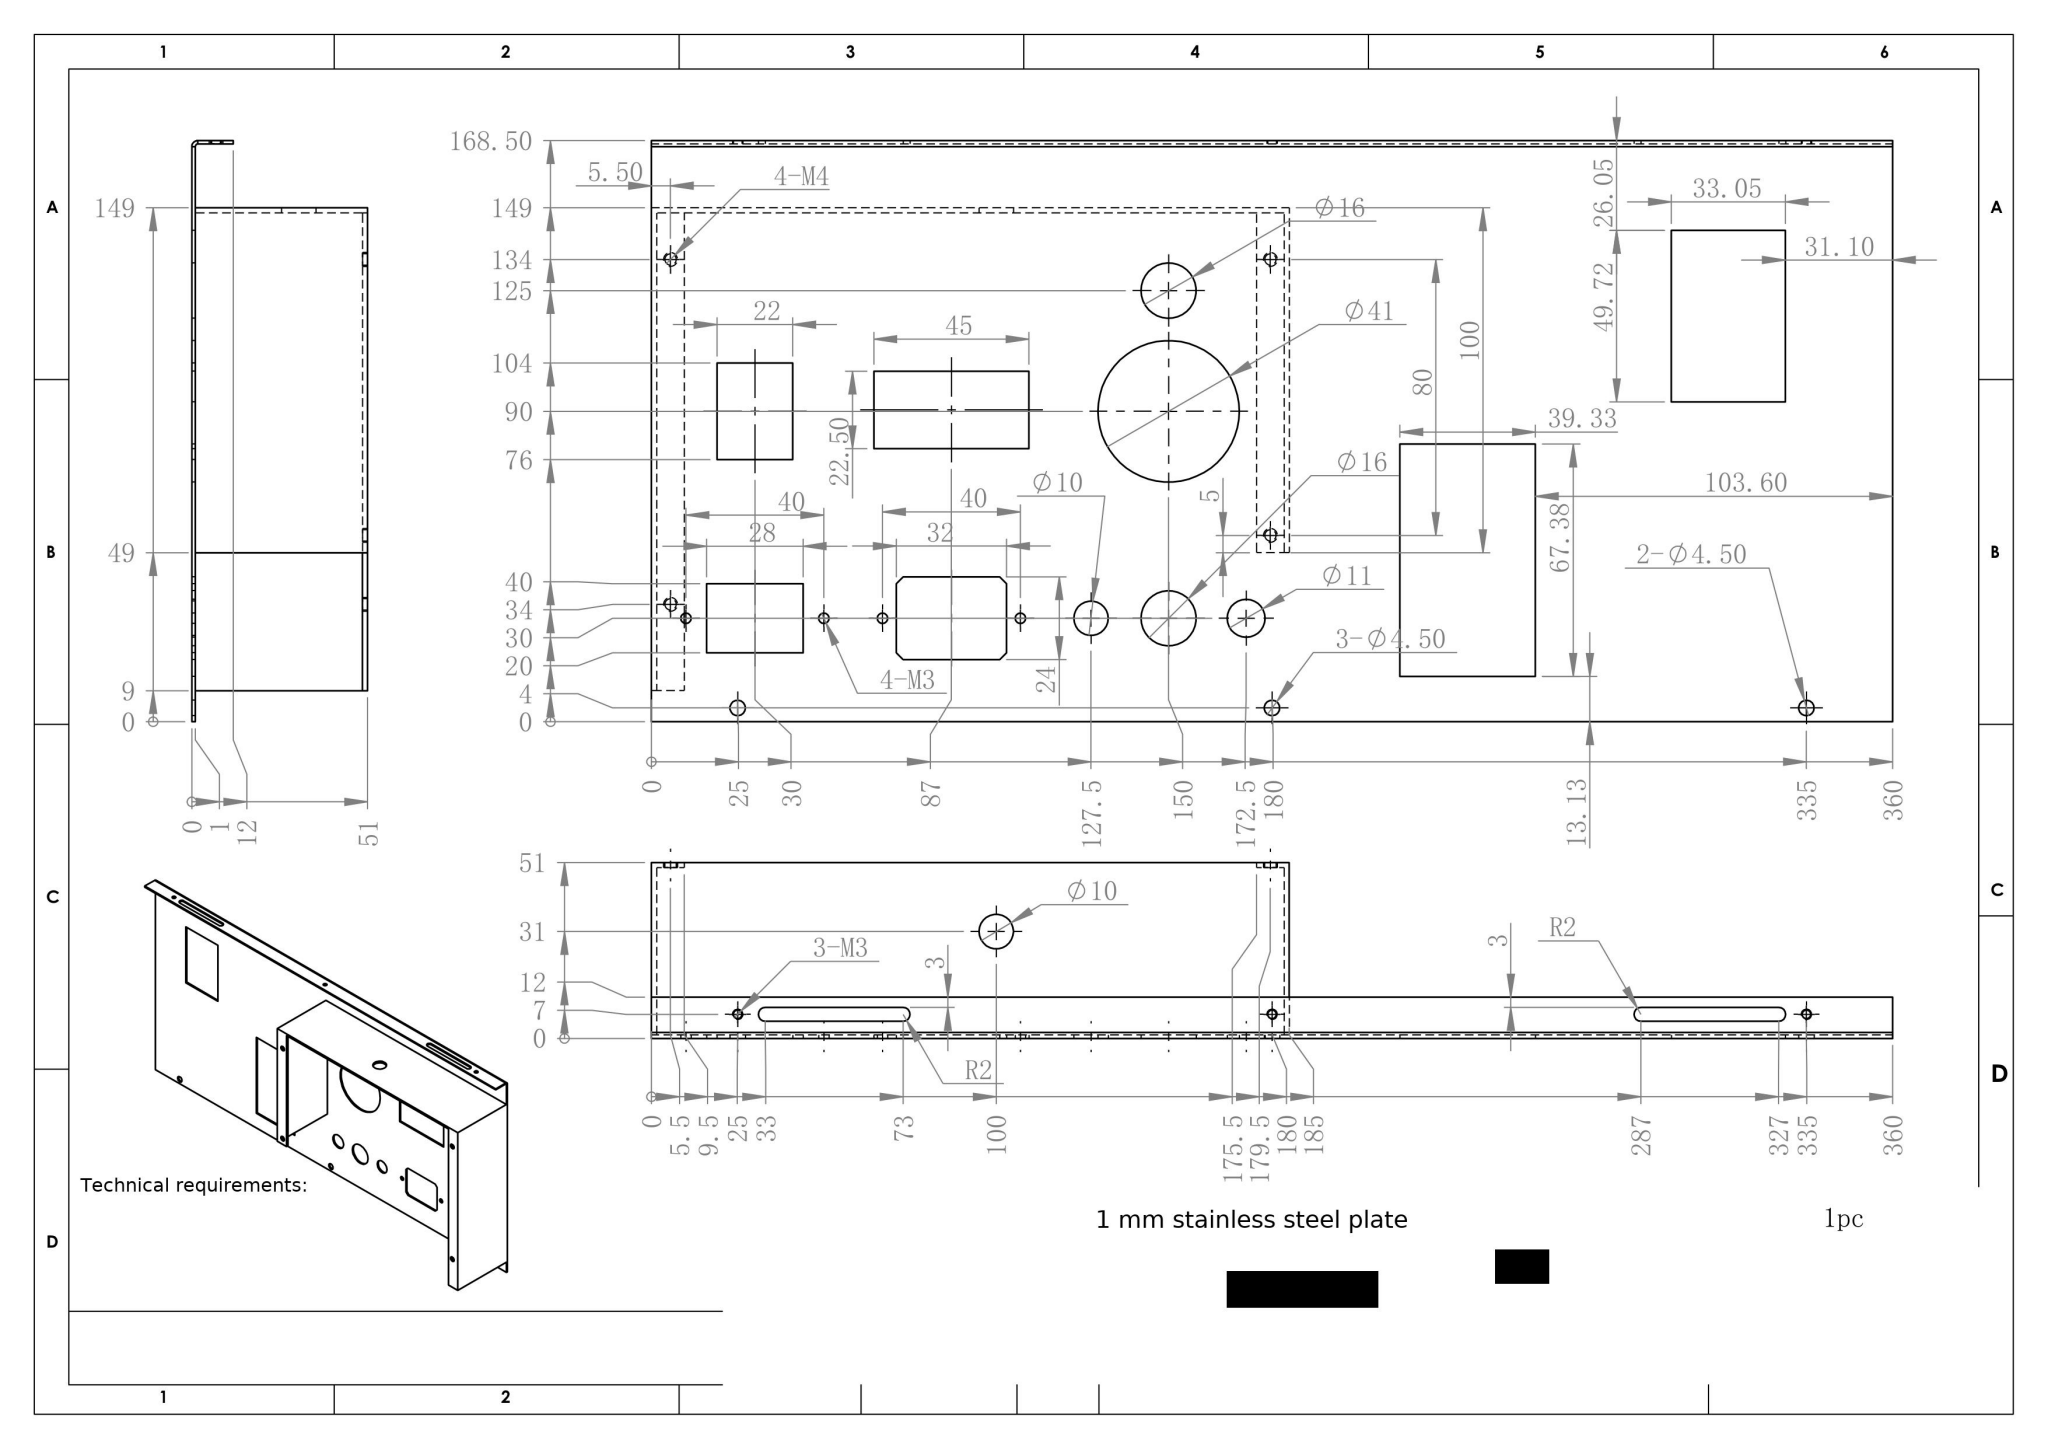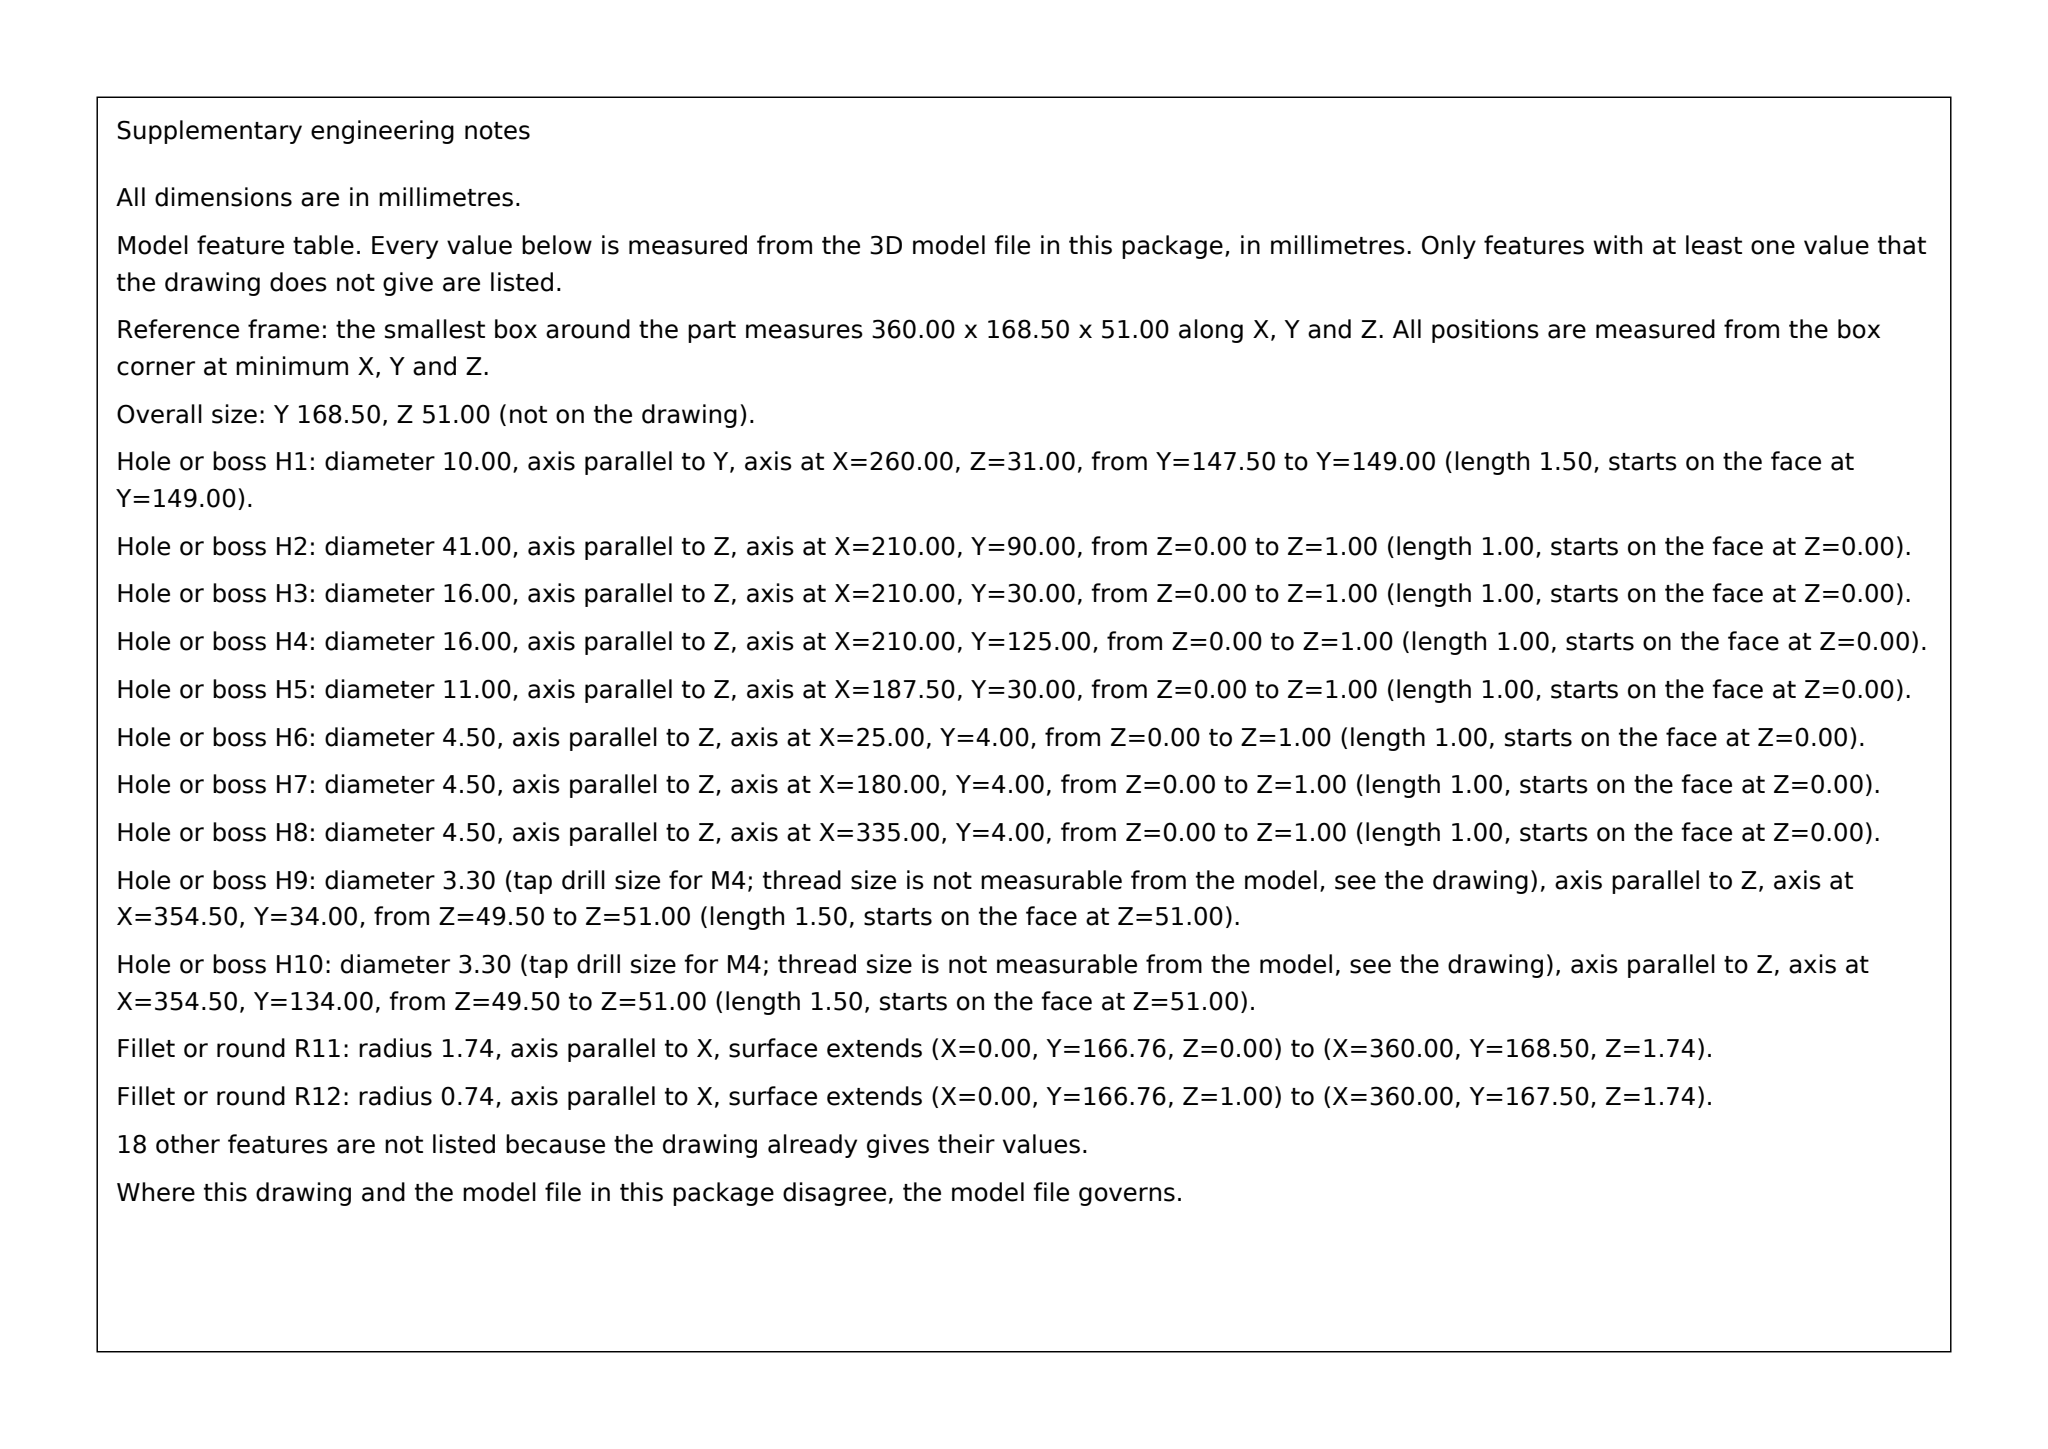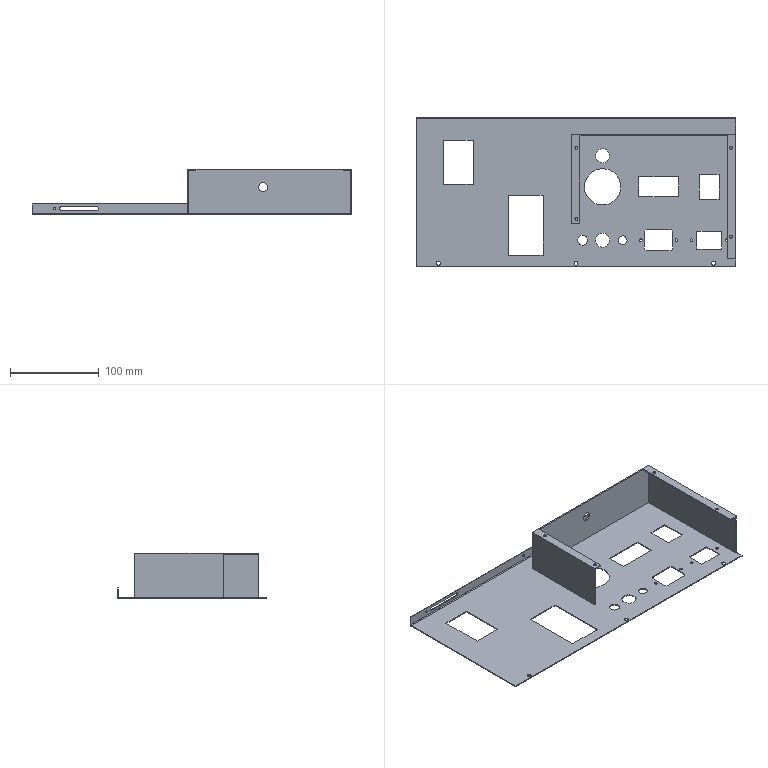Part | SolidWorks | mm | material 1 mm stainless steel plate | 1 solid | 102 faces | box 360 x 168.5 x 51 mm | volume 89180 mm3 | plane 56 | cylinder 46 | commonest cylinder face diameters 3.3 x8 3 x8 2.5 x6 4.5 x6 10 x4 16 x4 4 x4 41 x2